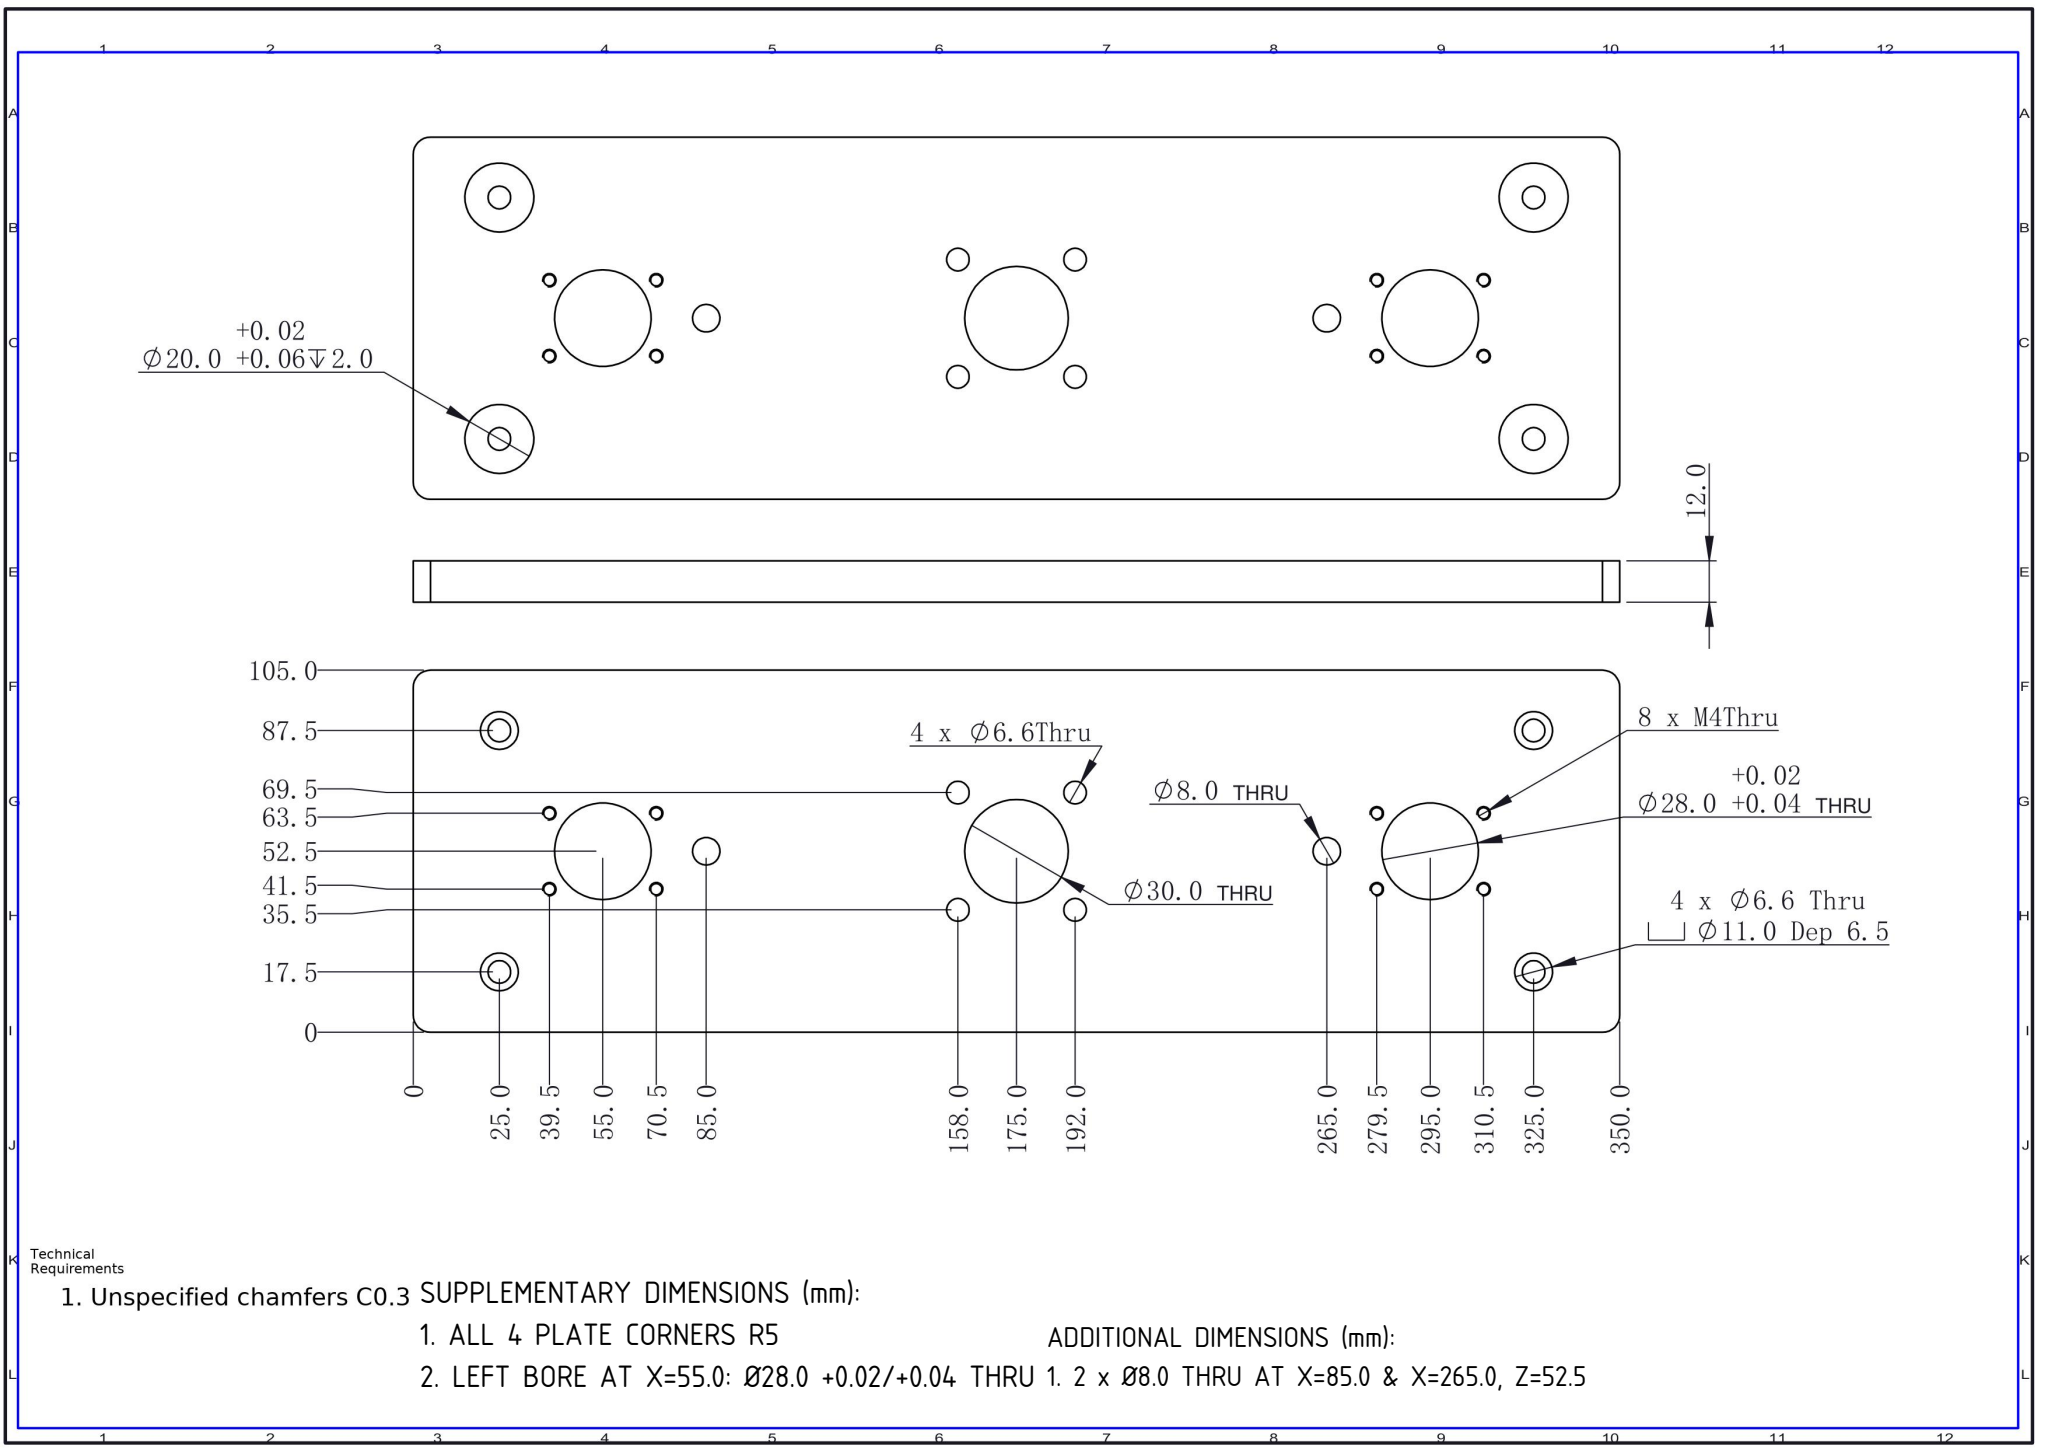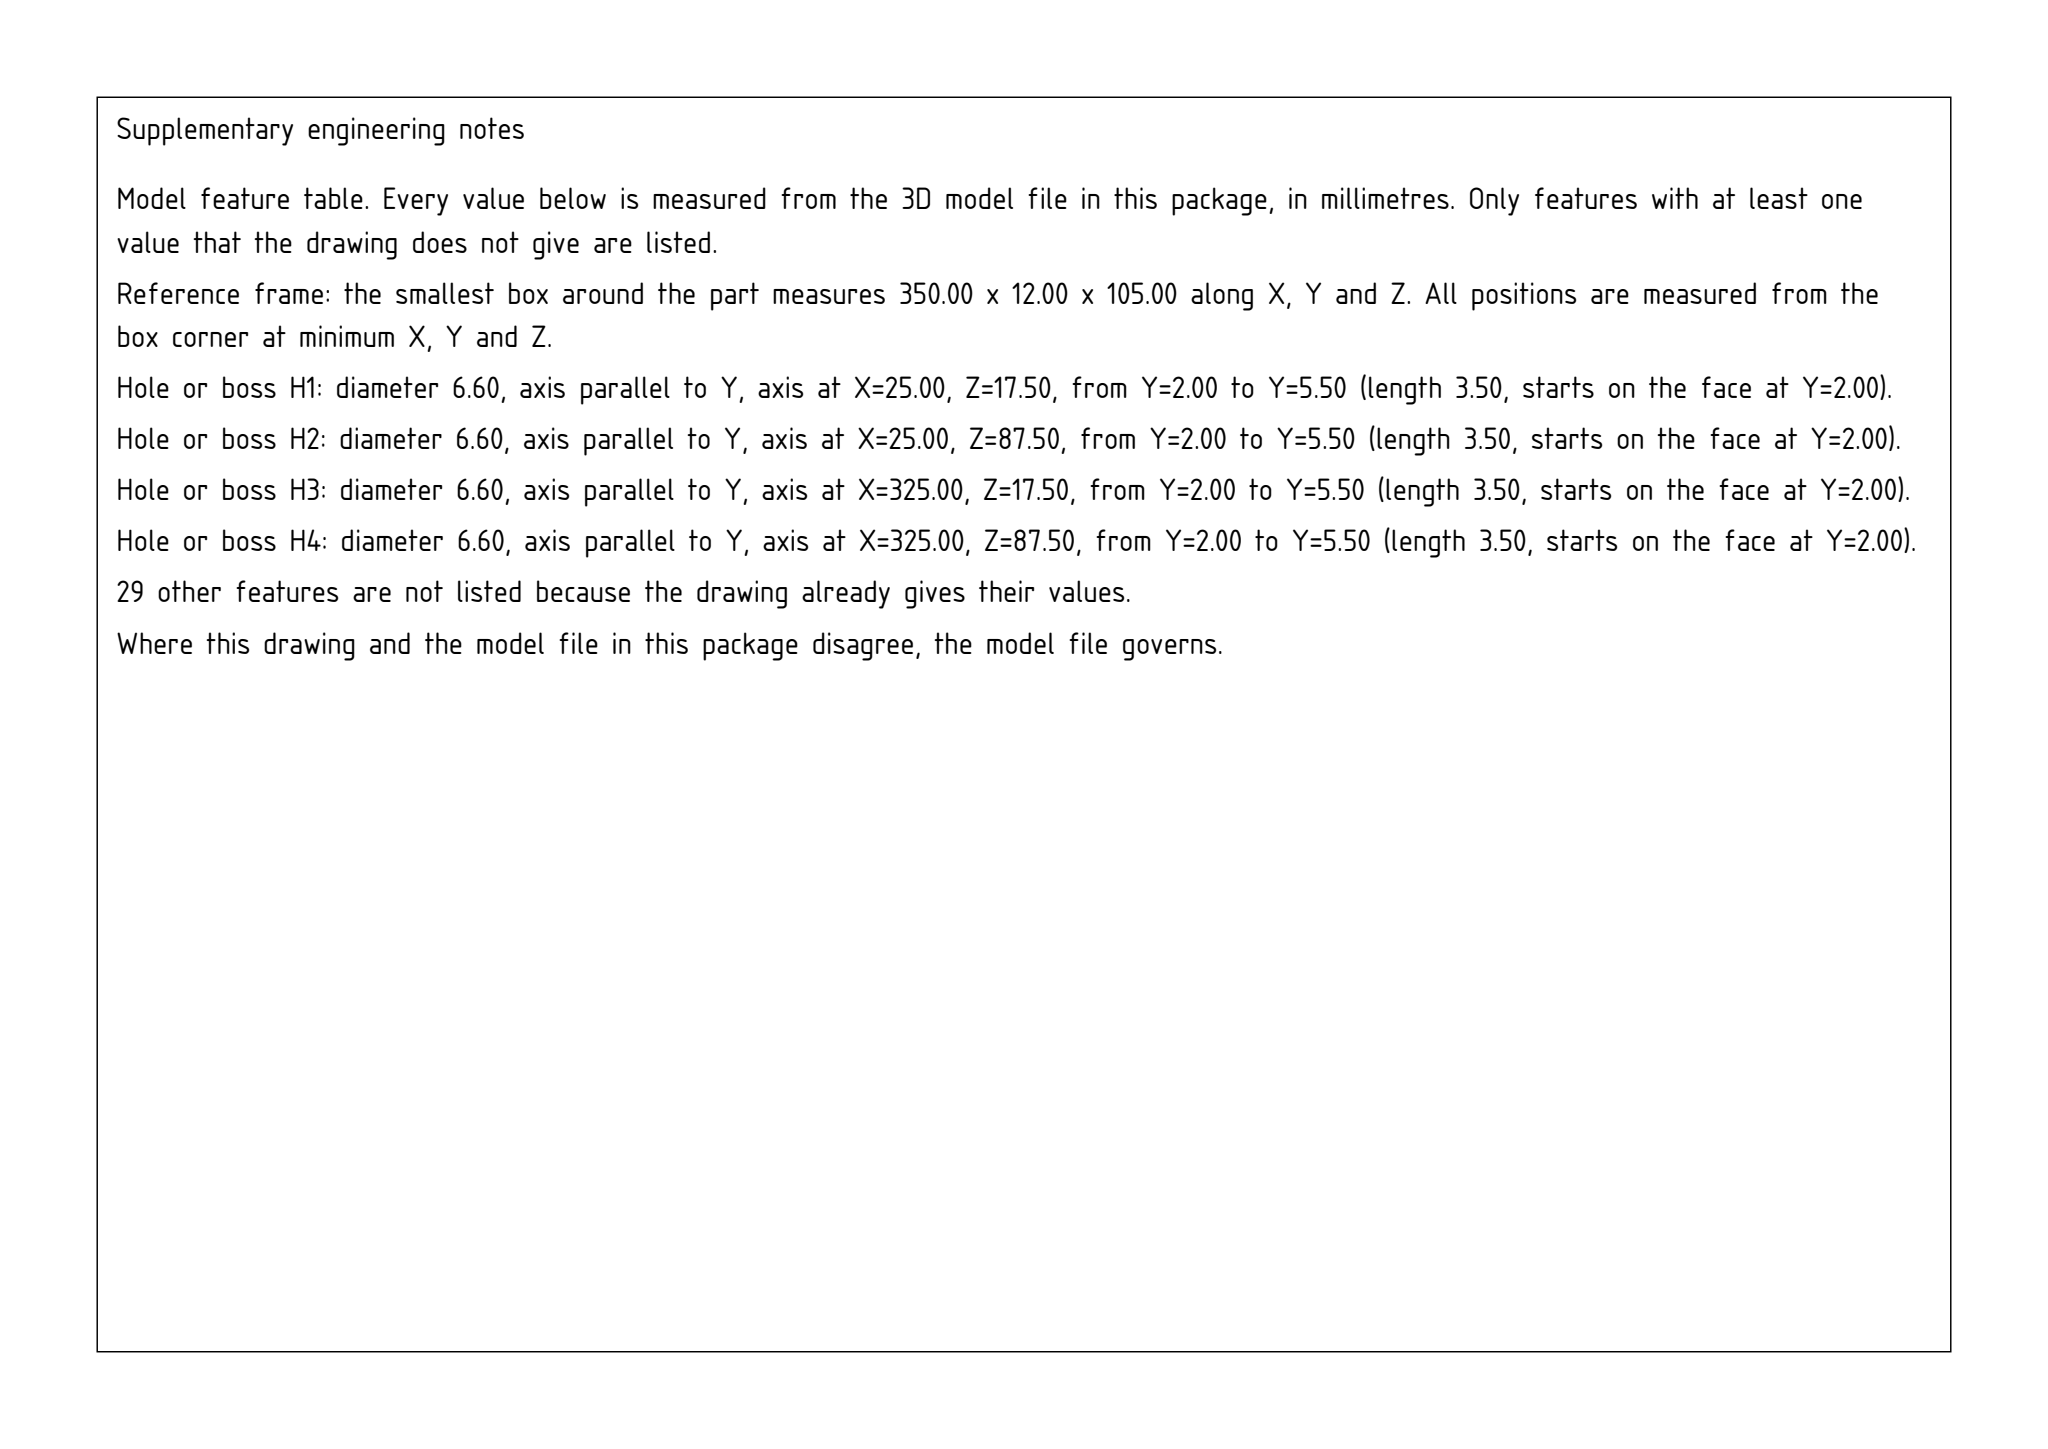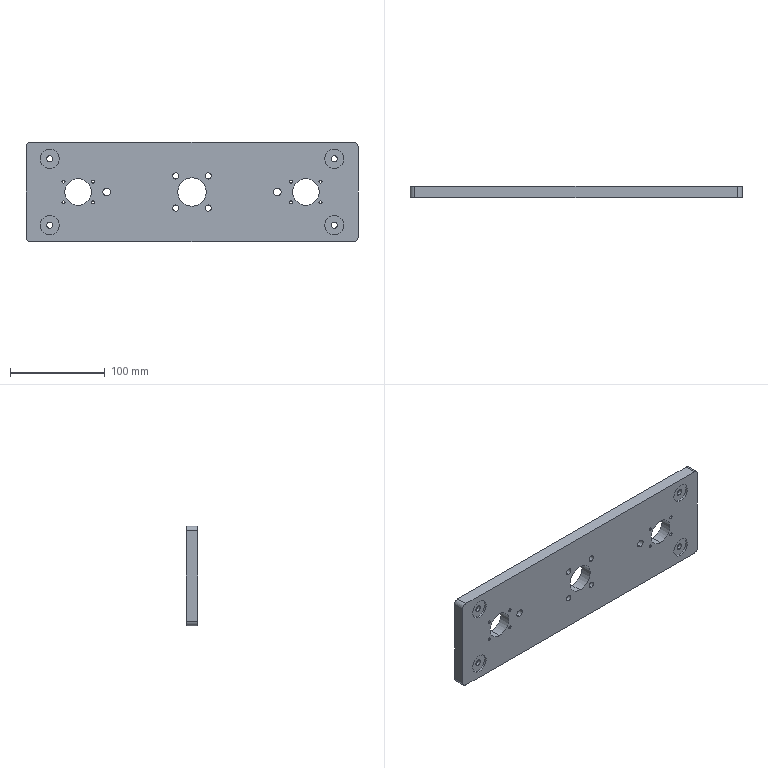Part | SolidWorks | mm | 1 solid | 76 faces | box 350 x 12 x 105 mm | volume 408349 mm3 | cylinder 62 | plane 14 | commonest cylinder face diameters 3.3 x16 6.6 x16 20 x8 11 x8 8 x4 28 x4 10 x4 30 x2